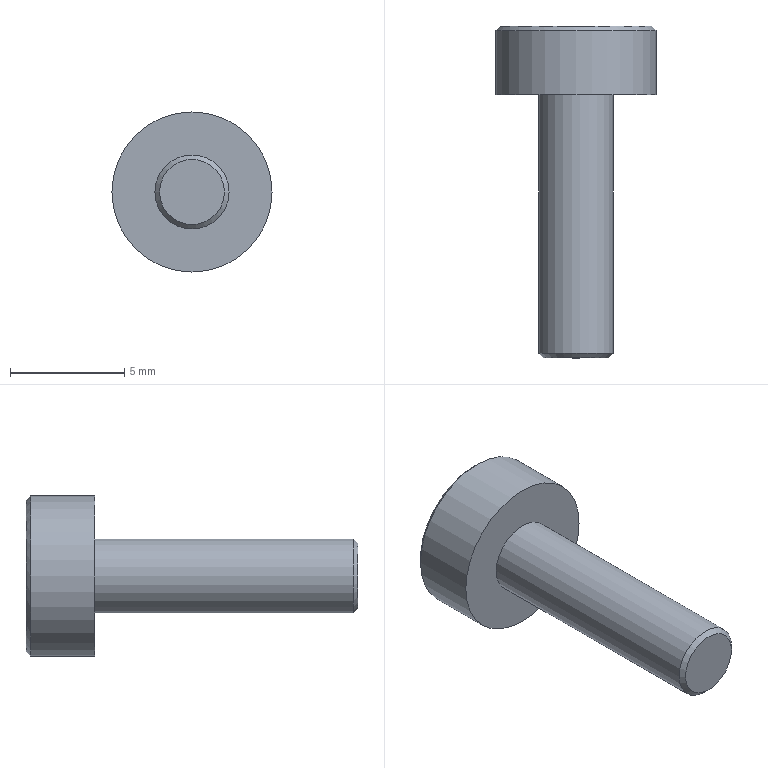Component | NX | HEX_CAP_SCREW_3 | 1 solid | 20 faces | volume 175 mm3 | plane 10 | cylinder 8 | cone 2 | commonest cylinder face diameters 2 x6 3.242 x1 7 x1